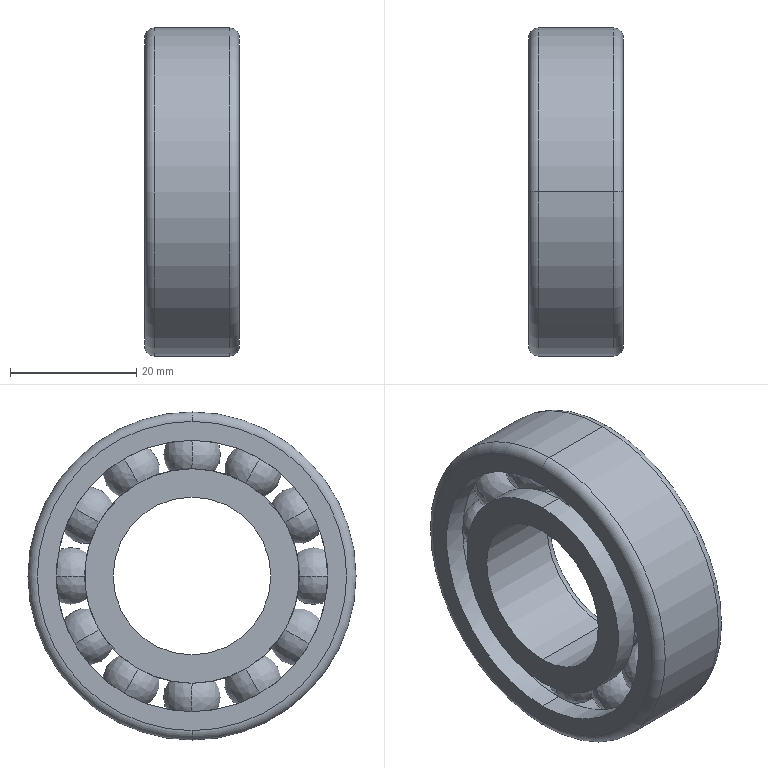Component | SolidWorks | 000504Y000006205-1 | 1 solid | 82 faces | volume 17719 mm3 | torus 42 | sphere 24 | cylinder 12 | plane 4 | commonest cylinder face diameters 43 x4 34 x4 52 x2 25 x2